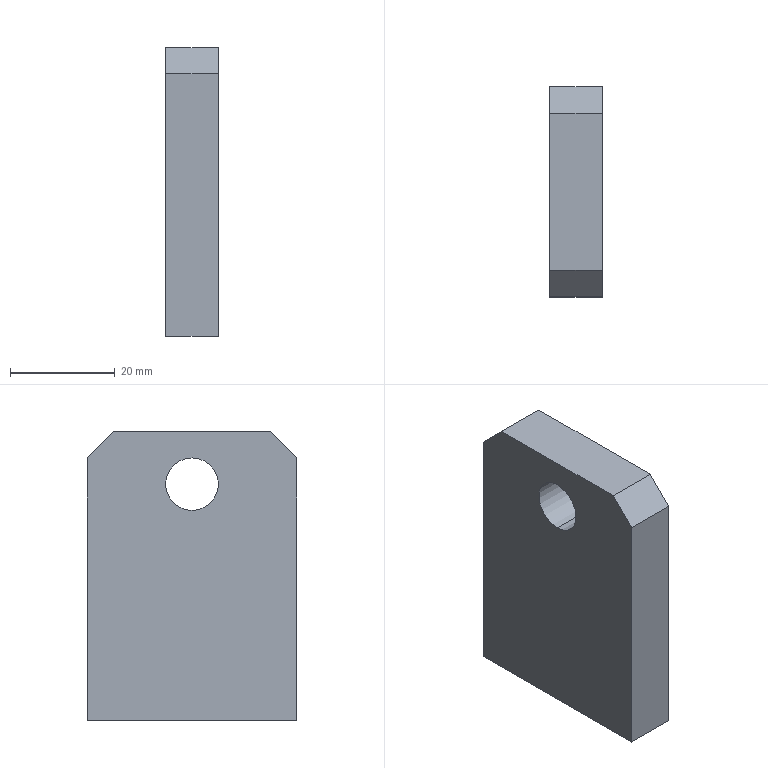Component | SolidWorks | 06-1 | 1 solid | 10 faces | box 10 x 40 x 55 mm | volume 20965 mm3 | plane 8 | cylinder 2 | commonest cylinder face diameters 10 x2
build123d program:
from build123d import *

# Parameters (mm, degrees)
SKETCH1_W           = 55
SKETCH1_H           = 40
SKETCH1_R           = 5
BOSS_EXTRUDE1_DEPTH = 10
CHAMFER1_SIZE       = 5


with BuildPart() as part:
    # Sketch1 → Boss-Extrude1 (new body)
    with BuildSketch(Plane(origin=(-180, 0, -160), x_dir=(0, 0, -1), z_dir=(1, 0, 0))):
        with Locations((-175.5, 210)):
            Rectangle(SKETCH1_W, SKETCH1_H)
        with Locations((-193, 210)):
            Circle(SKETCH1_R, mode=Mode.SUBTRACT)
    extrude(amount=-BOSS_EXTRUDE1_DEPTH)

    # Chamfer1
    chamfer1_edges = [part.edges().sort_by_distance(p)[0] for p in [
        (-185, 230, 43),
        (-185, 190, 43),
    ]]
    chamfer(chamfer1_edges, length=CHAMFER1_SIZE)


solid = part.part

# Placed as in the assembly
solid = solid.moved(Location((0, 0, 6), (0, 0, 0)))
STEP:
#1=COLOUR_RGB('',0.7922,0.8196,0.9333);
#2=FILL_AREA_STYLE_COLOUR('',#1);
#3=FILL_AREA_STYLE('',(#2));
#4=SURFACE_STYLE_FILL_AREA(#3);
#5=SURFACE_SIDE_STYLE('',(#4));
#6=SURFACE_STYLE_USAGE(.BOTH.,#5);
#7=PRESENTATION_STYLE_ASSIGNMENT((#6));
#8=CARTESIAN_POINT('',(-7.48,8.268,1.732));
#9=VERTEX_POINT('',#8);
#10=CARTESIAN_POINT('',(-7.48,8.268,1.339));
#11=VERTEX_POINT('',#10);
#12=CARTESIAN_POINT('',(-7.48,8.268,1.535));
#13=DIRECTION('',(1.,0.,0.));
#14=DIRECTION('',(0.,0.,-1.));
#15=AXIS2_PLACEMENT_3D('',#12,#13,#14);
#16=CIRCLE('',#15,0.1969);
#17=EDGE_CURVE('',#9,#11,#16,.T.);
#18=ORIENTED_EDGE('',*,*,#17,.F.);
#19=CARTESIAN_POINT('',(-7.087,8.268,1.732));
#20=VERTEX_POINT('',#19);
#21=CARTESIAN_POINT('',(-7.48,8.268,1.732));
#22=DIRECTION('',(1.,0.,0.));
#23=VECTOR('',#22,39.37);
#24=LINE('',#21,#23);
#25=EDGE_CURVE('',#9,#20,#24,.T.);
#26=ORIENTED_EDGE('',*,*,#25,.T.);
#27=CARTESIAN_POINT('',(-7.087,8.268,1.339));
#28=VERTEX_POINT('',#27);
#29=CARTESIAN_POINT('',(-7.087,8.268,1.535));
#30=DIRECTION('',(1.,0.,0.));
#31=DIRECTION('',(0.,0.,-1.));
#32=AXIS2_PLACEMENT_3D('',#29,#30,#31);
#33=CIRCLE('',#32,0.1969);
#34=EDGE_CURVE('',#20,#28,#33,.T.);
#35=ORIENTED_EDGE('',*,*,#34,.T.);
#36=CARTESIAN_POINT('',(-7.48,8.268,1.339));
#37=DIRECTION('',(1.,0.,0.));
#38=VECTOR('',#37,39.37);
#39=LINE('',#36,#38);
#40=EDGE_CURVE('',#11,#28,#39,.T.);
#41=ORIENTED_EDGE('',*,*,#40,.F.);
#42=EDGE_LOOP('',(#18,#26,#35,#41));
#43=FACE_OUTER_BOUND('',#42,.T.);
#44=CARTESIAN_POINT('',(-7.48,8.268,1.535));
#45=DIRECTION('',(1.,0.,0.));
#46=DIRECTION('',(0.,0.,-1.));
#47=AXIS2_PLACEMENT_3D('',#44,#45,#46);
#48=CYLINDRICAL_SURFACE('',#47,0.1969);
#49=ADVANCED_FACE('',(#43),#48,.F.);
#50=CARTESIAN_POINT('',(-7.48,8.858,1.929));
#51=VERTEX_POINT('',#50);
#52=CARTESIAN_POINT('',(-7.48,7.677,1.929));
#53=VERTEX_POINT('',#52);
#54=CARTESIAN_POINT('',(-7.48,9.055,1.929));
#55=DIRECTION('',(0.,-1.,0.));
#56=VECTOR('',#55,39.37);
#57=LINE('',#54,#56);
#58=EDGE_CURVE('',#51,#53,#57,.T.);
#59=ORIENTED_EDGE('',*,*,#58,.T.);
#60=CARTESIAN_POINT('',(-7.087,7.677,1.929));
#61=VERTEX_POINT('',#60);
#62=CARTESIAN_POINT('',(-7.48,7.677,1.929));
#63=DIRECTION('',(1.,0.,0.));
#64=VECTOR('',#63,39.37);
#65=LINE('',#62,#64);
#66=EDGE_CURVE('',#53,#61,#65,.T.);
#67=ORIENTED_EDGE('',*,*,#66,.T.);
#68=CARTESIAN_POINT('',(-7.087,8.858,1.929));
#69=VERTEX_POINT('',#68);
#70=CARTESIAN_POINT('',(-7.087,9.055,1.929));
#71=DIRECTION('',(0.,-1.,0.));
#72=VECTOR('',#71,39.37);
#73=LINE('',#70,#72);
#74=EDGE_CURVE('',#69,#61,#73,.T.);
#75=ORIENTED_EDGE('',*,*,#74,.F.);
#76=CARTESIAN_POINT('',(-7.48,8.858,1.929));
#77=DIRECTION('',(-1.,0.,0.));
#78=VECTOR('',#77,39.37);
#79=LINE('',#76,#78);
#80=EDGE_CURVE('',#69,#51,#79,.T.);
#81=ORIENTED_EDGE('',*,*,#80,.T.);
#82=EDGE_LOOP('',(#59,#67,#75,#81));
#83=FACE_OUTER_BOUND('',#82,.T.);
#84=CARTESIAN_POINT('',(-7.48,9.055,1.929));
#85=DIRECTION('',(0.,0.,1.));
#86=DIRECTION('',(1.,0.,0.));
#87=AXIS2_PLACEMENT_3D('',#84,#85,#86);
#88=PLANE('',#87);
#89=ADVANCED_FACE('',(#83),#88,.T.);
#90=CARTESIAN_POINT('',(-7.48,9.055,-0.2362));
#91=VERTEX_POINT('',#90);
#92=CARTESIAN_POINT('',(-7.48,9.055,1.732));
#93=VERTEX_POINT('',#92);
#94=CARTESIAN_POINT('',(-7.48,9.055,1.929));
#95=DIRECTION('',(0.,0.,1.));
#96=VECTOR('',#95,39.37);
#97=LINE('',#94,#96);
#98=EDGE_CURVE('',#91,#93,#97,.T.);
#99=ORIENTED_EDGE('',*,*,#98,.T.);
#100=CARTESIAN_POINT('',(-7.087,9.055,1.732));
#101=VERTEX_POINT('',#100);
#102=CARTESIAN_POINT('',(-7.48,9.055,1.732));
#103=DIRECTION('',(1.,0.,0.));
#104=VECTOR('',#103,39.37);
#105=LINE('',#102,#104);
#106=EDGE_CURVE('',#93,#101,#105,.T.);
#107=ORIENTED_EDGE('',*,*,#106,.T.);
#108=CARTESIAN_POINT('',(-7.087,9.055,-0.2362));
#109=VERTEX_POINT('',#108);
#110=CARTESIAN_POINT('',(-7.087,9.055,1.929));
#111=DIRECTION('',(0.,0.,1.));
#112=VECTOR('',#111,39.37);
#113=LINE('',#110,#112);
#114=EDGE_CURVE('',#109,#101,#113,.T.);
#115=ORIENTED_EDGE('',*,*,#114,.F.);
#116=CARTESIAN_POINT('',(-7.48,9.055,-0.2362));
#117=DIRECTION('',(1.,0.,0.));
#118=VECTOR('',#117,39.37);
#119=LINE('',#116,#118);
#120=EDGE_CURVE('',#91,#109,#119,.T.);
#121=ORIENTED_EDGE('',*,*,#120,.F.);
#122=EDGE_LOOP('',(#99,#107,#115,#121));
#123=FACE_OUTER_BOUND('',#122,.T.);
#124=CARTESIAN_POINT('',(-7.48,9.055,1.929));
#125=DIRECTION('',(0.,1.,0.));
#126=DIRECTION('',(0.,0.,1.));
#127=AXIS2_PLACEMENT_3D('',#124,#125,#126);
#128=PLANE('',#127);
#129=ADVANCED_FACE('',(#123),#128,.T.);
#130=CARTESIAN_POINT('',(-7.087,7.48,-0.2362));
#131=VERTEX_POINT('',#130);
#132=CARTESIAN_POINT('',(-7.087,9.055,-0.2362));
#133=DIRECTION('',(0.,1.,0.));
#134=VECTOR('',#133,39.37);
#135=LINE('',#132,#134);
#136=EDGE_CURVE('',#131,#109,#135,.T.);
#137=ORIENTED_EDGE('',*,*,#136,.F.);
#138=CARTESIAN_POINT('',(-7.48,7.48,-0.2362));
#139=VERTEX_POINT('',#138);
#140=CARTESIAN_POINT('',(-7.48,7.48,-0.2362));
#141=DIRECTION('',(1.,0.,0.));
#142=VECTOR('',#141,39.37);
#143=LINE('',#140,#142);
#144=EDGE_CURVE('',#139,#131,#143,.T.);
#145=ORIENTED_EDGE('',*,*,#144,.F.);
#146=CARTESIAN_POINT('',(-7.48,9.055,-0.2362));
#147=DIRECTION('',(0.,1.,0.));
#148=VECTOR('',#147,39.37);
#149=LINE('',#146,#148);
#150=EDGE_CURVE('',#139,#91,#149,.T.);
#151=ORIENTED_EDGE('',*,*,#150,.T.);
#152=ORIENTED_EDGE('',*,*,#120,.T.);
#153=EDGE_LOOP('',(#137,#145,#151,#152));
#154=FACE_OUTER_BOUND('',#153,.T.);
#155=CARTESIAN_POINT('',(-7.48,9.055,-0.2362));
#156=DIRECTION('',(0.,0.,-1.));
#157=DIRECTION('',(-1.,0.,0.));
#158=AXIS2_PLACEMENT_3D('',#155,#156,#157);
#159=PLANE('',#158);
#160=ADVANCED_FACE('',(#154),#159,.T.);
#161=CARTESIAN_POINT('',(-7.087,7.48,1.732));
#162=VERTEX_POINT('',#161);
#163=CARTESIAN_POINT('',(-7.087,7.48,1.929));
#164=DIRECTION('',(0.,0.,-1.));
#165=VECTOR('',#164,39.37);
#166=LINE('',#163,#165);
#167=EDGE_CURVE('',#162,#131,#166,.T.);
#168=ORIENTED_EDGE('',*,*,#167,.F.);
#169=CARTESIAN_POINT('',(-7.48,7.48,1.732));
#170=VERTEX_POINT('',#169);
#171=CARTESIAN_POINT('',(-7.48,7.48,1.732));
#172=DIRECTION('',(-1.,0.,0.));
#173=VECTOR('',#172,39.37);
#174=LINE('',#171,#173);
#175=EDGE_CURVE('',#162,#170,#174,.T.);
#176=ORIENTED_EDGE('',*,*,#175,.T.);
#177=CARTESIAN_POINT('',(-7.48,7.48,1.929));
#178=DIRECTION('',(0.,0.,-1.));
#179=VECTOR('',#178,39.37);
#180=LINE('',#177,#179);
#181=EDGE_CURVE('',#170,#139,#180,.T.);
#182=ORIENTED_EDGE('',*,*,#181,.T.);
#183=ORIENTED_EDGE('',*,*,#144,.T.);
#184=EDGE_LOOP('',(#168,#176,#182,#183));
#185=FACE_OUTER_BOUND('',#184,.T.);
#186=CARTESIAN_POINT('',(-7.48,7.48,1.929));
#187=DIRECTION('',(0.,-1.,0.));
#188=DIRECTION('',(0.,0.,-1.));
#189=AXIS2_PLACEMENT_3D('',#186,#187,#188);
#190=PLANE('',#189);
#191=ADVANCED_FACE('',(#185),#190,.T.);
#192=CARTESIAN_POINT('',(-7.48,8.268,1.535));
#193=DIRECTION('',(1.,0.,0.));
#194=DIRECTION('',(0.,0.,-1.));
#195=AXIS2_PLACEMENT_3D('',#192,#193,#194);
#196=CIRCLE('',#195,0.1969);
#197=EDGE_CURVE('',#11,#9,#196,.T.);
#198=ORIENTED_EDGE('',*,*,#197,.T.);
#199=ORIENTED_EDGE('',*,*,#17,.T.);
#200=EDGE_LOOP('',(#198,#199));
#201=FACE_BOUND('',#200,.T.);
#202=ORIENTED_EDGE('',*,*,#181,.F.);
#203=CARTESIAN_POINT('',(-7.48,7.677,1.929));
#204=DIRECTION('',(0.,0.7071,0.7071));
#205=VECTOR('',#204,39.37);
#206=LINE('',#203,#205);
#207=EDGE_CURVE('',#170,#53,#206,.T.);
#208=ORIENTED_EDGE('',*,*,#207,.T.);
#209=ORIENTED_EDGE('',*,*,#58,.F.);
#210=CARTESIAN_POINT('',(-7.48,9.055,1.732));
#211=DIRECTION('',(0.,0.7071,-0.7071));
#212=VECTOR('',#211,39.37);
#213=LINE('',#210,#212);
#214=EDGE_CURVE('',#51,#93,#213,.T.);
#215=ORIENTED_EDGE('',*,*,#214,.T.);
#216=ORIENTED_EDGE('',*,*,#98,.F.);
#217=ORIENTED_EDGE('',*,*,#150,.F.);
#218=EDGE_LOOP('',(#202,#208,#209,#215,#216,#217));
#219=FACE_OUTER_BOUND('',#218,.T.);
#220=CARTESIAN_POINT('',(-7.48,0.,0.2362));
#221=DIRECTION('',(1.,0.,0.));
#222=DIRECTION('',(0.,0.,-1.));
#223=AXIS2_PLACEMENT_3D('',#220,#221,#222);
#224=PLANE('',#223);
#225=ADVANCED_FACE('',(#201,#219),#224,.F.);
#226=CARTESIAN_POINT('',(-7.087,8.268,1.535));
#227=DIRECTION('',(1.,0.,0.));
#228=DIRECTION('',(0.,0.,-1.));
#229=AXIS2_PLACEMENT_3D('',#226,#227,#228);
#230=CIRCLE('',#229,0.1969);
#231=EDGE_CURVE('',#28,#20,#230,.T.);
#232=ORIENTED_EDGE('',*,*,#231,.F.);
#233=ORIENTED_EDGE('',*,*,#34,.F.);
#234=EDGE_LOOP('',(#232,#233));
#235=FACE_BOUND('',#234,.T.);
#236=ORIENTED_EDGE('',*,*,#74,.T.);
#237=CARTESIAN_POINT('',(-7.087,2.992,-2.756));
#238=DIRECTION('',(0.,-0.7071,-0.7071));
#239=VECTOR('',#238,39.37);
#240=LINE('',#237,#239);
#241=EDGE_CURVE('',#61,#162,#240,.T.);
#242=ORIENTED_EDGE('',*,*,#241,.T.);
#243=ORIENTED_EDGE('',*,*,#167,.T.);
#244=ORIENTED_EDGE('',*,*,#136,.T.);
#245=ORIENTED_EDGE('',*,*,#114,.T.);
#246=CARTESIAN_POINT('',(-7.087,5.276,5.512));
#247=DIRECTION('',(0.,-0.7071,0.7071));
#248=VECTOR('',#247,39.37);
#249=LINE('',#246,#248);
#250=EDGE_CURVE('',#101,#69,#249,.T.);
#251=ORIENTED_EDGE('',*,*,#250,.T.);
#252=EDGE_LOOP('',(#236,#242,#243,#244,#245,#251));
#253=FACE_OUTER_BOUND('',#252,.T.);
#254=CARTESIAN_POINT('',(-7.087,0.,0.2362));
#255=DIRECTION('',(1.,0.,0.));
#256=DIRECTION('',(0.,0.,-1.));
#257=AXIS2_PLACEMENT_3D('',#254,#255,#256);
#258=PLANE('',#257);
#259=ADVANCED_FACE('',(#235,#253),#258,.T.);
#260=ORIENTED_EDGE('',*,*,#25,.F.);
#261=ORIENTED_EDGE('',*,*,#197,.F.);
#262=ORIENTED_EDGE('',*,*,#40,.T.);
#263=ORIENTED_EDGE('',*,*,#231,.T.);
#264=EDGE_LOOP('',(#260,#261,#262,#263));
#265=FACE_OUTER_BOUND('',#264,.T.);
#266=CARTESIAN_POINT('',(-7.48,8.268,1.535));
#267=DIRECTION('',(1.,0.,0.));
#268=DIRECTION('',(0.,0.,-1.));
#269=AXIS2_PLACEMENT_3D('',#266,#267,#268);
#270=CYLINDRICAL_SURFACE('',#269,0.1969);
#271=ADVANCED_FACE('',(#265),#270,.F.);
#272=ORIENTED_EDGE('',*,*,#207,.F.);
#273=ORIENTED_EDGE('',*,*,#175,.F.);
#274=ORIENTED_EDGE('',*,*,#241,.F.);
#275=ORIENTED_EDGE('',*,*,#66,.F.);
#276=EDGE_LOOP('',(#272,#273,#274,#275));
#277=FACE_OUTER_BOUND('',#276,.T.);
#278=CARTESIAN_POINT('',(-7.48,7.677,1.929));
#279=DIRECTION('',(0.,0.7071,-0.7071));
#280=DIRECTION('',(1.,0.,0.));
#281=AXIS2_PLACEMENT_3D('',#278,#279,#280);
#282=PLANE('',#281);
#283=ADVANCED_FACE('',(#277),#282,.F.);
#284=ORIENTED_EDGE('',*,*,#214,.F.);
#285=ORIENTED_EDGE('',*,*,#80,.F.);
#286=ORIENTED_EDGE('',*,*,#250,.F.);
#287=ORIENTED_EDGE('',*,*,#106,.F.);
#288=EDGE_LOOP('',(#284,#285,#286,#287));
#289=FACE_OUTER_BOUND('',#288,.T.);
#290=CARTESIAN_POINT('',(-7.48,9.055,1.732));
#291=DIRECTION('',(0.,-0.7071,-0.7071));
#292=DIRECTION('',(1.,0.,0.));
#293=AXIS2_PLACEMENT_3D('',#290,#291,#292);
#294=PLANE('',#293);
#295=ADVANCED_FACE('',(#289),#294,.F.);
#296=CLOSED_SHELL('',(#49,#89,#129,#160,#191,#225,#259,#271,#283,#295));
#297=MANIFOLD_SOLID_BREP('',#296);
#298=STYLED_ITEM('',(#7),#297);
#299=(LENGTH_UNIT()NAMED_UNIT(*)SI_UNIT($,.METRE.));
#300=LENGTH_MEASURE_WITH_UNIT(LENGTH_MEASURE(0.0254),#299);
#301=DIMENSIONAL_EXPONENTS(1.,0.,0.,0.,0.,0.,0.);
#302=(CONVERSION_BASED_UNIT('',#300)LENGTH_UNIT()NAMED_UNIT(#301));
#303=UNCERTAINTY_MEASURE_WITH_UNIT(LENGTH_MEASURE(0.00001),#302,'','');
#304=(NAMED_UNIT(*)PLANE_ANGLE_UNIT()SI_UNIT($,.RADIAN.));
#305=(NAMED_UNIT(*)SI_UNIT($,.STERADIAN.)SOLID_ANGLE_UNIT());
#306=(GEOMETRIC_REPRESENTATION_CONTEXT(3)GLOBAL_UNCERTAINTY_ASSIGNED_CONTEXT((#303))GLOBAL_UNIT_ASSIGNED_CONTEXT((#302,#304,#305))REPRESENTATION_CONTEXT('',''));
#307=MECHANICAL_DESIGN_GEOMETRIC_PRESENTATION_REPRESENTATION('',(#298),#306);
#308=CARTESIAN_POINT('',(0.,0.,0.));
#309=DIRECTION('',(0.,0.,1.));
#310=DIRECTION('',(1.,0.,0.));
#311=AXIS2_PLACEMENT_3D('',#308,#309,#310);
#312=(LENGTH_UNIT()NAMED_UNIT(*)SI_UNIT($,.METRE.));
#313=LENGTH_MEASURE_WITH_UNIT(LENGTH_MEASURE(0.0254),#312);
#314=DIMENSIONAL_EXPONENTS(1.,0.,0.,0.,0.,0.,0.);
#315=(CONVERSION_BASED_UNIT('',#313)LENGTH_UNIT()NAMED_UNIT(#314));
#316=UNCERTAINTY_MEASURE_WITH_UNIT(LENGTH_MEASURE(0.00001),#315,'','');
#317=(NAMED_UNIT(*)PLANE_ANGLE_UNIT()SI_UNIT($,.RADIAN.));
#318=(NAMED_UNIT(*)SI_UNIT($,.STERADIAN.)SOLID_ANGLE_UNIT());
#319=(GEOMETRIC_REPRESENTATION_CONTEXT(3)GLOBAL_UNCERTAINTY_ASSIGNED_CONTEXT((#316))GLOBAL_UNIT_ASSIGNED_CONTEXT((#315,#317,#318))REPRESENTATION_CONTEXT('',''));
#320=ADVANCED_BREP_SHAPE_REPRESENTATION('',(#297,#311),#319);
#321=PRESENTATION_LAYER_ASSIGNMENT('','',(#298));